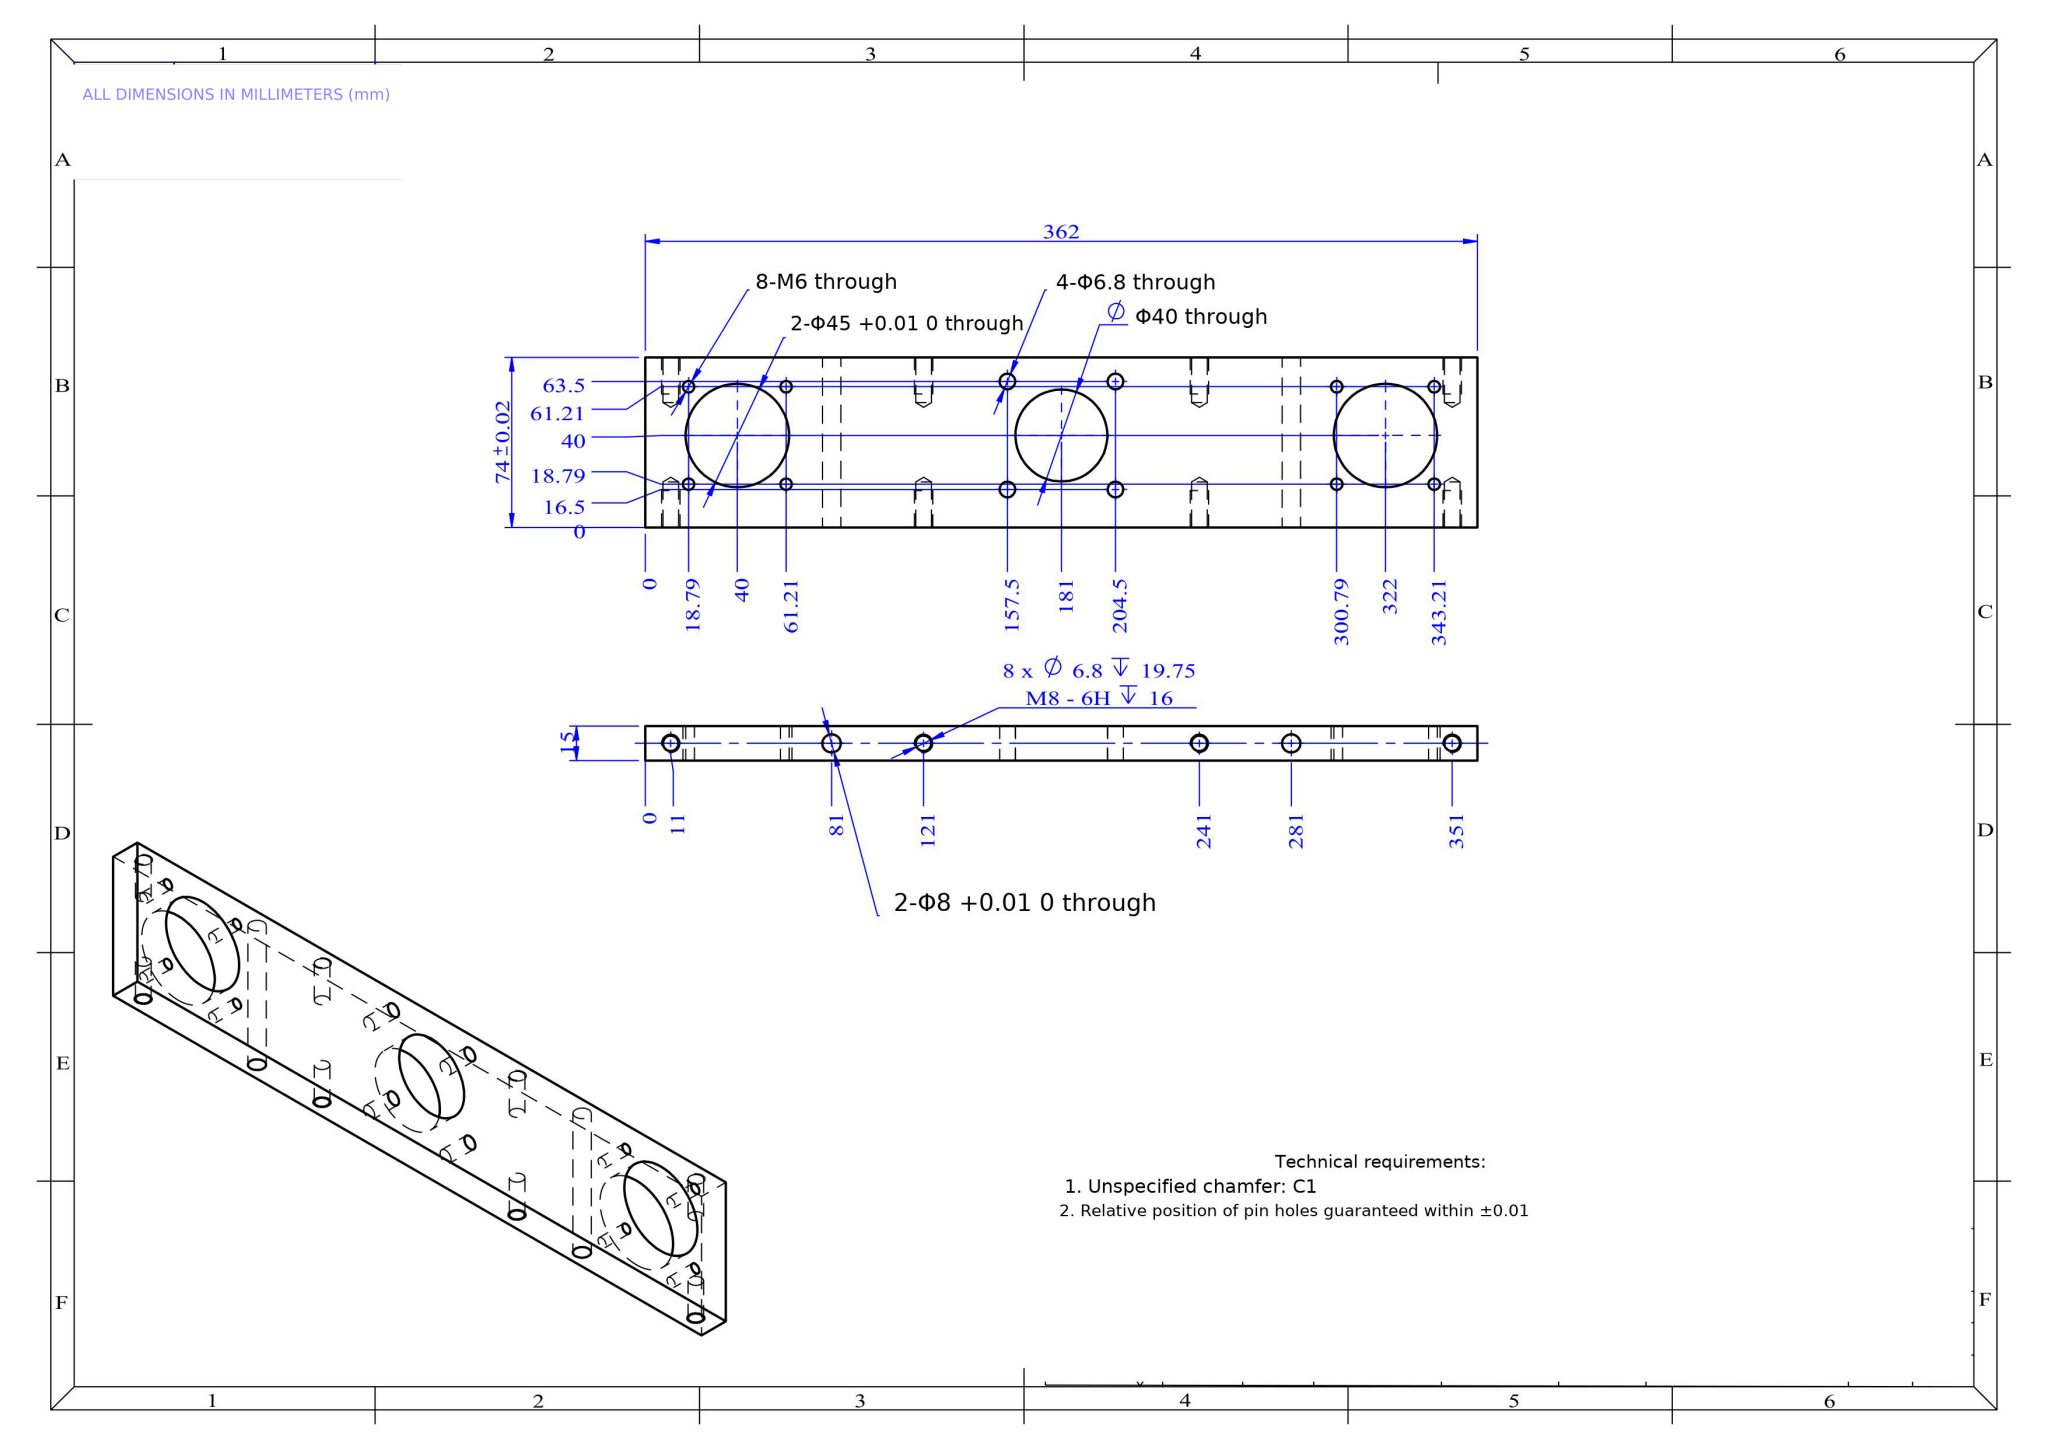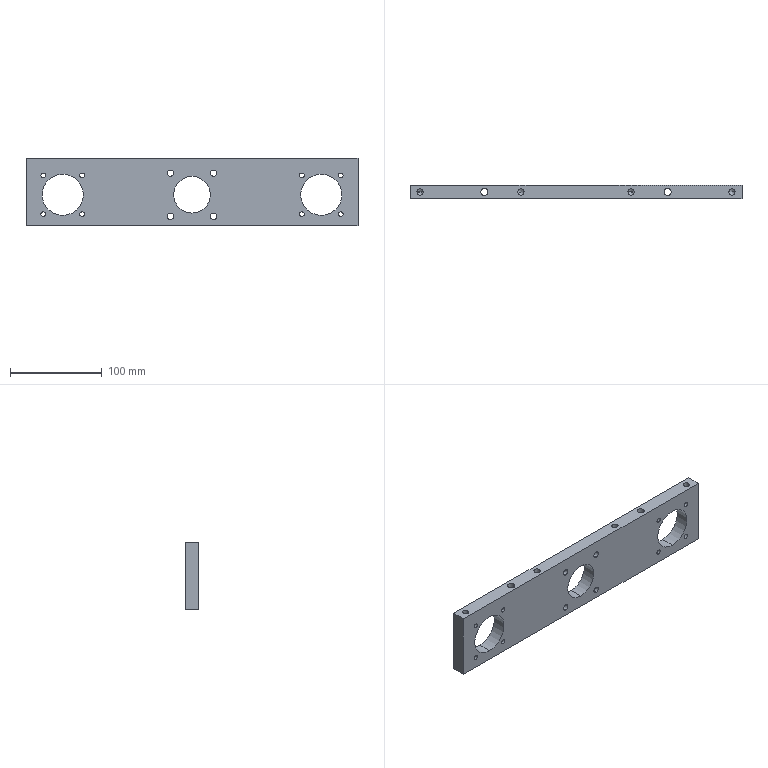Part | NX | mm | 1 solid | 72 faces | box 362 x 15 x 74 mm | volume 317347 mm3 | cylinder 50 | cone 16 | plane 6 | commonest cylinder face diameters 6.8 x24 5 x16 8 x4 45 x4 40 x2